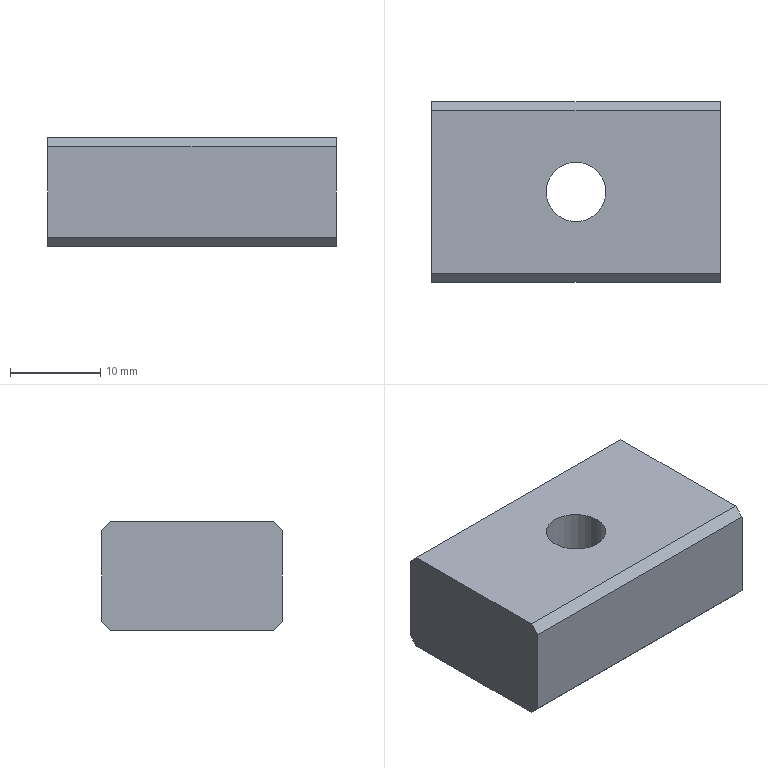Component | NX | LOCATING_KEY | 1 solid | 13 faces | box 32 x 20 x 12 mm | volume 6792 mm3 | plane 11 | cylinder 2 | commonest cylinder face diameters 6.6 x1 11 x1
STEP:
#1=CARTESIAN_POINT('',(0.,0.,0.));
#2=DIRECTION('',(0.,0.,1.));
#3=DIRECTION('',(1.,0.,0.));
#4=AXIS2_PLACEMENT_3D('',#1,#2,#3);
#5=CARTESIAN_POINT('',(250.,10.,-50.));
#6=VERTEX_POINT('',#5);
#7=CARTESIAN_POINT('',(250.,10.,-60.));
#8=VERTEX_POINT('',#7);
#9=CARTESIAN_POINT('',(250.,10.,-49.));
#10=DIRECTION('',(0.,0.,-1.));
#11=VECTOR('',#10,1.);
#12=LINE('',#9,#11);
#13=CARTESIAN_POINT('',(250.,10.,-49.));
#14=DIRECTION('',(1.,0.,0.));
#15=DIRECTION('',(0.,0.,-1.));
#16=AXIS2_PLACEMENT_3D('',#13,#14,#15);
#17=PLANE('',#16);
#18=CARTESIAN_POINT('',(0.,0.));
#19=DIRECTION('',(1.,0.));
#20=VECTOR('',#19,1.);
#21=LINE('',#18,#20);
#22=(GEOMETRIC_REPRESENTATION_CONTEXT(2)PARAMETRIC_REPRESENTATION_CONTEXT()REPRESENTATION_CONTEXT('',''));
#23=DEFINITIONAL_REPRESENTATION('',(#21),#22);
#24=PCURVE('',#17,#23);
#25=CARTESIAN_POINT('',(282.,10.,-49.));
#26=DIRECTION('',(0.,-1.,0.));
#27=DIRECTION('',(0.,0.,-1.));
#28=AXIS2_PLACEMENT_3D('',#25,#26,#27);
#29=PLANE('',#28);
#30=CARTESIAN_POINT('',(0.,-32.));
#31=DIRECTION('',(1.,0.));
#32=VECTOR('',#31,1.);
#33=LINE('',#30,#32);
#34=(GEOMETRIC_REPRESENTATION_CONTEXT(2)PARAMETRIC_REPRESENTATION_CONTEXT()REPRESENTATION_CONTEXT('',''));
#35=DEFINITIONAL_REPRESENTATION('',(#33),#34);
#36=PCURVE('',#29,#35);
#37=SURFACE_CURVE('',#12,(#24,#36),.PCURVE_S1.);
#38=EDGE_CURVE('',#6,#8,#37,.T.);
#39=ORIENTED_EDGE('',*,*,#38,.T.);
#40=CARTESIAN_POINT('',(250.,9.,-61.));
#41=VERTEX_POINT('',#40);
#42=CARTESIAN_POINT('',(250.,10.,-60.));
#43=DIRECTION('',(0.,-0.7071,-0.7071));
#44=VECTOR('',#43,1.);
#45=LINE('',#42,#44);
#46=CARTESIAN_POINT('',(11.,0.));
#47=DIRECTION('',(0.7071,-0.7071));
#48=VECTOR('',#47,1.);
#49=LINE('',#46,#48);
#50=(GEOMETRIC_REPRESENTATION_CONTEXT(2)PARAMETRIC_REPRESENTATION_CONTEXT()REPRESENTATION_CONTEXT('',''));
#51=DEFINITIONAL_REPRESENTATION('',(#49),#50);
#52=PCURVE('',#17,#51);
#53=CARTESIAN_POINT('',(282.,10.,-60.));
#54=DIRECTION('',(0.,-0.7071,0.7071));
#55=DIRECTION('',(-1.,0.,0.));
#56=AXIS2_PLACEMENT_3D('',#53,#54,#55);
#57=PLANE('',#56);
#58=CARTESIAN_POINT('',(32.,0.));
#59=DIRECTION('',(0.,1.));
#60=VECTOR('',#59,1.);
#61=LINE('',#58,#60);
#62=(GEOMETRIC_REPRESENTATION_CONTEXT(2)PARAMETRIC_REPRESENTATION_CONTEXT()REPRESENTATION_CONTEXT('',''));
#63=DEFINITIONAL_REPRESENTATION('',(#61),#62);
#64=PCURVE('',#57,#63);
#65=SURFACE_CURVE('',#45,(#52,#64),.PCURVE_S1.);
#66=EDGE_CURVE('',#8,#41,#65,.T.);
#67=ORIENTED_EDGE('',*,*,#66,.T.);
#68=CARTESIAN_POINT('',(250.,-9.,-61.));
#69=VERTEX_POINT('',#68);
#70=CARTESIAN_POINT('',(250.,10.,-61.));
#71=DIRECTION('',(0.,-1.,0.));
#72=VECTOR('',#71,1.);
#73=LINE('',#70,#72);
#74=CARTESIAN_POINT('',(12.,0.));
#75=DIRECTION('',(0.,-1.));
#76=VECTOR('',#75,1.);
#77=LINE('',#74,#76);
#78=(GEOMETRIC_REPRESENTATION_CONTEXT(2)PARAMETRIC_REPRESENTATION_CONTEXT()REPRESENTATION_CONTEXT('',''));
#79=DEFINITIONAL_REPRESENTATION('',(#77),#78);
#80=PCURVE('',#17,#79);
#81=CARTESIAN_POINT('',(266.,-0.,-61.));
#82=DIRECTION('',(0.,0.,1.));
#83=DIRECTION('',(1.,0.,0.));
#84=AXIS2_PLACEMENT_3D('',#81,#82,#83);
#85=PLANE('',#84);
#86=CARTESIAN_POINT('',(-16.,10.));
#87=DIRECTION('',(0.,-1.));
#88=VECTOR('',#87,1.);
#89=LINE('',#86,#88);
#90=(GEOMETRIC_REPRESENTATION_CONTEXT(2)PARAMETRIC_REPRESENTATION_CONTEXT()REPRESENTATION_CONTEXT('',''));
#91=DEFINITIONAL_REPRESENTATION('',(#89),#90);
#92=PCURVE('',#85,#91);
#93=SURFACE_CURVE('',#73,(#80,#92),.PCURVE_S1.);
#94=EDGE_CURVE('',#41,#69,#93,.T.);
#95=ORIENTED_EDGE('',*,*,#94,.T.);
#96=CARTESIAN_POINT('',(250.,-10.,-60.));
#97=VERTEX_POINT('',#96);
#98=CARTESIAN_POINT('',(250.,-10.,-60.));
#99=DIRECTION('',(0.,-0.7071,0.7071));
#100=VECTOR('',#99,1.);
#101=LINE('',#98,#100);
#102=CARTESIAN_POINT('',(11.,-20.));
#103=DIRECTION('',(-0.7071,-0.7071));
#104=VECTOR('',#103,1.);
#105=LINE('',#102,#104);
#106=(GEOMETRIC_REPRESENTATION_CONTEXT(2)PARAMETRIC_REPRESENTATION_CONTEXT()REPRESENTATION_CONTEXT('',''));
#107=DEFINITIONAL_REPRESENTATION('',(#105),#106);
#108=PCURVE('',#17,#107);
#109=CARTESIAN_POINT('',(250.,-10.,-60.));
#110=DIRECTION('',(0.,0.7071,0.7071));
#111=DIRECTION('',(1.,0.,0.));
#112=AXIS2_PLACEMENT_3D('',#109,#110,#111);
#113=PLANE('',#112);
#114=CARTESIAN_POINT('',(0.,0.));
#115=DIRECTION('',(0.,-1.));
#116=VECTOR('',#115,1.);
#117=LINE('',#114,#116);
#118=(GEOMETRIC_REPRESENTATION_CONTEXT(2)PARAMETRIC_REPRESENTATION_CONTEXT()REPRESENTATION_CONTEXT('',''));
#119=DEFINITIONAL_REPRESENTATION('',(#117),#118);
#120=PCURVE('',#113,#119);
#121=SURFACE_CURVE('',#101,(#108,#120),.PCURVE_S1.);
#122=EDGE_CURVE('',#69,#97,#121,.T.);
#123=ORIENTED_EDGE('',*,*,#122,.T.);
#124=CARTESIAN_POINT('',(250.,-10.,-50.));
#125=VERTEX_POINT('',#124);
#126=CARTESIAN_POINT('',(250.,-10.,-49.));
#127=DIRECTION('',(0.,0.,-1.));
#128=VECTOR('',#127,1.);
#129=LINE('',#126,#128);
#130=CARTESIAN_POINT('',(0.,-20.));
#131=DIRECTION('',(1.,0.));
#132=VECTOR('',#131,1.);
#133=LINE('',#130,#132);
#134=(GEOMETRIC_REPRESENTATION_CONTEXT(2)PARAMETRIC_REPRESENTATION_CONTEXT()REPRESENTATION_CONTEXT('',''));
#135=DEFINITIONAL_REPRESENTATION('',(#133),#134);
#136=PCURVE('',#17,#135);
#137=CARTESIAN_POINT('',(250.,-10.,-49.));
#138=DIRECTION('',(0.,1.,0.));
#139=DIRECTION('',(0.,0.,1.));
#140=AXIS2_PLACEMENT_3D('',#137,#138,#139);
#141=PLANE('',#140);
#142=CARTESIAN_POINT('',(0.,0.));
#143=DIRECTION('',(-1.,0.));
#144=VECTOR('',#143,1.);
#145=LINE('',#142,#144);
#146=(GEOMETRIC_REPRESENTATION_CONTEXT(2)PARAMETRIC_REPRESENTATION_CONTEXT()REPRESENTATION_CONTEXT('',''));
#147=DEFINITIONAL_REPRESENTATION('',(#145),#146);
#148=PCURVE('',#141,#147);
#149=SURFACE_CURVE('',#129,(#136,#148),.PCURVE_S1.);
#150=EDGE_CURVE('',#125,#97,#149,.T.);
#151=ORIENTED_EDGE('',*,*,#150,.F.);
#152=CARTESIAN_POINT('',(250.,-9.,-49.));
#153=VERTEX_POINT('',#152);
#154=CARTESIAN_POINT('',(250.,-9.,-49.));
#155=DIRECTION('',(0.,0.7071,0.7071));
#156=VECTOR('',#155,1.);
#157=LINE('',#154,#156);
#158=CARTESIAN_POINT('',(0.,-19.));
#159=DIRECTION('',(-0.7071,0.7071));
#160=VECTOR('',#159,1.);
#161=LINE('',#158,#160);
#162=(GEOMETRIC_REPRESENTATION_CONTEXT(2)PARAMETRIC_REPRESENTATION_CONTEXT()REPRESENTATION_CONTEXT('',''));
#163=DEFINITIONAL_REPRESENTATION('',(#161),#162);
#164=PCURVE('',#17,#163);
#165=CARTESIAN_POINT('',(266.,-9.,-49.));
#166=DIRECTION('',(0.,-0.7071,0.7071));
#167=DIRECTION('',(-1.,0.,0.));
#168=AXIS2_PLACEMENT_3D('',#165,#166,#167);
#169=PLANE('',#168);
#170=CARTESIAN_POINT('',(16.,0.));
#171=DIRECTION('',(0.,-1.));
#172=VECTOR('',#171,1.);
#173=LINE('',#170,#172);
#174=(GEOMETRIC_REPRESENTATION_CONTEXT(2)PARAMETRIC_REPRESENTATION_CONTEXT()REPRESENTATION_CONTEXT('',''));
#175=DEFINITIONAL_REPRESENTATION('',(#173),#174);
#176=PCURVE('',#169,#175);
#177=SURFACE_CURVE('',#157,(#164,#176),.PCURVE_S1.);
#178=EDGE_CURVE('',#125,#153,#177,.T.);
#179=ORIENTED_EDGE('',*,*,#178,.T.);
#180=CARTESIAN_POINT('',(250.,9.,-49.));
#181=VERTEX_POINT('',#180);
#182=CARTESIAN_POINT('',(250.,10.,-49.));
#183=DIRECTION('',(0.,-1.,0.));
#184=VECTOR('',#183,1.);
#185=LINE('',#182,#184);
#186=CARTESIAN_POINT('',(0.,0.));
#187=DIRECTION('',(0.,-1.));
#188=VECTOR('',#187,1.);
#189=LINE('',#186,#188);
#190=(GEOMETRIC_REPRESENTATION_CONTEXT(2)PARAMETRIC_REPRESENTATION_CONTEXT()REPRESENTATION_CONTEXT('',''));
#191=DEFINITIONAL_REPRESENTATION('',(#189),#190);
#192=PCURVE('',#17,#191);
#193=CARTESIAN_POINT('',(266.,-0.,-49.));
#194=DIRECTION('',(0.,0.,1.));
#195=DIRECTION('',(1.,0.,0.));
#196=AXIS2_PLACEMENT_3D('',#193,#194,#195);
#197=PLANE('',#196);
#198=CARTESIAN_POINT('',(-16.,10.));
#199=DIRECTION('',(0.,-1.));
#200=VECTOR('',#199,1.);
#201=LINE('',#198,#200);
#202=(GEOMETRIC_REPRESENTATION_CONTEXT(2)PARAMETRIC_REPRESENTATION_CONTEXT()REPRESENTATION_CONTEXT('',''));
#203=DEFINITIONAL_REPRESENTATION('',(#201),#202);
#204=PCURVE('',#197,#203);
#205=SURFACE_CURVE('',#185,(#192,#204),.PCURVE_S1.);
#206=EDGE_CURVE('',#181,#153,#205,.T.);
#207=ORIENTED_EDGE('',*,*,#206,.F.);
#208=CARTESIAN_POINT('',(250.,9.,-49.));
#209=DIRECTION('',(0.,0.7071,-0.7071));
#210=VECTOR('',#209,1.);
#211=LINE('',#208,#210);
#212=CARTESIAN_POINT('',(0.,-1.));
#213=DIRECTION('',(0.7071,0.7071));
#214=VECTOR('',#213,1.);
#215=LINE('',#212,#214);
#216=(GEOMETRIC_REPRESENTATION_CONTEXT(2)PARAMETRIC_REPRESENTATION_CONTEXT()REPRESENTATION_CONTEXT('',''));
#217=DEFINITIONAL_REPRESENTATION('',(#215),#216);
#218=PCURVE('',#17,#217);
#219=CARTESIAN_POINT('',(266.,9.,-49.));
#220=DIRECTION('',(0.,0.7071,0.7071));
#221=DIRECTION('',(1.,0.,0.));
#222=AXIS2_PLACEMENT_3D('',#219,#220,#221);
#223=PLANE('',#222);
#224=CARTESIAN_POINT('',(-16.,0.));
#225=DIRECTION('',(0.,1.));
#226=VECTOR('',#225,1.);
#227=LINE('',#224,#226);
#228=(GEOMETRIC_REPRESENTATION_CONTEXT(2)PARAMETRIC_REPRESENTATION_CONTEXT()REPRESENTATION_CONTEXT('',''));
#229=DEFINITIONAL_REPRESENTATION('',(#227),#228);
#230=PCURVE('',#223,#229);
#231=SURFACE_CURVE('',#211,(#218,#230),.PCURVE_S1.);
#232=EDGE_CURVE('',#181,#6,#231,.T.);
#233=ORIENTED_EDGE('',*,*,#232,.T.);
#234=EDGE_LOOP('',(#39,#67,#95,#123,#151,#179,#207,#233));
#235=FACE_BOUND('',#234,.T.);
#236=ADVANCED_FACE('',(#235),#17,.F.);
#237=ORIENTED_EDGE('',*,*,#150,.T.);
#238=CARTESIAN_POINT('',(282.,-10.,-60.));
#239=VERTEX_POINT('',#238);
#240=CARTESIAN_POINT('',(250.,-10.,-60.));
#241=DIRECTION('',(1.,0.,0.));
#242=VECTOR('',#241,1.);
#243=LINE('',#240,#242);
#244=CARTESIAN_POINT('',(-11.,0.));
#245=DIRECTION('',(0.,1.));
#246=VECTOR('',#245,1.);
#247=LINE('',#244,#246);
#248=(GEOMETRIC_REPRESENTATION_CONTEXT(2)PARAMETRIC_REPRESENTATION_CONTEXT()REPRESENTATION_CONTEXT('',''));
#249=DEFINITIONAL_REPRESENTATION('',(#247),#248);
#250=PCURVE('',#141,#249);
#251=CARTESIAN_POINT('',(0.,0.));
#252=DIRECTION('',(1.,0.));
#253=VECTOR('',#252,1.);
#254=LINE('',#251,#253);
#255=(GEOMETRIC_REPRESENTATION_CONTEXT(2)PARAMETRIC_REPRESENTATION_CONTEXT()REPRESENTATION_CONTEXT('',''));
#256=DEFINITIONAL_REPRESENTATION('',(#254),#255);
#257=PCURVE('',#113,#256);
#258=SURFACE_CURVE('',#243,(#250,#257),.PCURVE_S1.);
#259=EDGE_CURVE('',#97,#239,#258,.T.);
#260=ORIENTED_EDGE('',*,*,#259,.T.);
#261=CARTESIAN_POINT('',(282.,-10.,-50.));
#262=VERTEX_POINT('',#261);
#263=CARTESIAN_POINT('',(282.,-10.,-49.));
#264=DIRECTION('',(0.,0.,-1.));
#265=VECTOR('',#264,1.);
#266=LINE('',#263,#265);
#267=CARTESIAN_POINT('',(0.,32.));
#268=DIRECTION('',(-1.,0.));
#269=VECTOR('',#268,1.);
#270=LINE('',#267,#269);
#271=(GEOMETRIC_REPRESENTATION_CONTEXT(2)PARAMETRIC_REPRESENTATION_CONTEXT()REPRESENTATION_CONTEXT('',''));
#272=DEFINITIONAL_REPRESENTATION('',(#270),#271);
#273=PCURVE('',#141,#272);
#274=CARTESIAN_POINT('',(282.,-10.,-49.));
#275=DIRECTION('',(-1.,0.,0.));
#276=DIRECTION('',(0.,0.,1.));
#277=AXIS2_PLACEMENT_3D('',#274,#275,#276);
#278=PLANE('',#277);
#279=CARTESIAN_POINT('',(0.,0.));
#280=DIRECTION('',(-1.,0.));
#281=VECTOR('',#280,1.);
#282=LINE('',#279,#281);
#283=(GEOMETRIC_REPRESENTATION_CONTEXT(2)PARAMETRIC_REPRESENTATION_CONTEXT()REPRESENTATION_CONTEXT('',''));
#284=DEFINITIONAL_REPRESENTATION('',(#282),#283);
#285=PCURVE('',#278,#284);
#286=SURFACE_CURVE('',#266,(#273,#285),.PCURVE_S1.);
#287=EDGE_CURVE('',#262,#239,#286,.T.);
#288=ORIENTED_EDGE('',*,*,#287,.F.);
#289=CARTESIAN_POINT('',(250.,-10.,-50.));
#290=DIRECTION('',(-1.,0.,0.));
#291=VECTOR('',#290,1.);
#292=LINE('',#289,#291);
#293=CARTESIAN_POINT('',(-1.,0.));
#294=DIRECTION('',(0.,-1.));
#295=VECTOR('',#294,1.);
#296=LINE('',#293,#295);
#297=(GEOMETRIC_REPRESENTATION_CONTEXT(2)PARAMETRIC_REPRESENTATION_CONTEXT()REPRESENTATION_CONTEXT('',''));
#298=DEFINITIONAL_REPRESENTATION('',(#296),#297);
#299=PCURVE('',#141,#298);
#300=CARTESIAN_POINT('',(16.,1.414));
#301=DIRECTION('',(1.,0.));
#302=VECTOR('',#301,1.);
#303=LINE('',#300,#302);
#304=(GEOMETRIC_REPRESENTATION_CONTEXT(2)PARAMETRIC_REPRESENTATION_CONTEXT()REPRESENTATION_CONTEXT('',''));
#305=DEFINITIONAL_REPRESENTATION('',(#303),#304);
#306=PCURVE('',#169,#305);
#307=SURFACE_CURVE('',#292,(#299,#306),.PCURVE_S1.);
#308=EDGE_CURVE('',#262,#125,#307,.T.);
#309=ORIENTED_EDGE('',*,*,#308,.T.);
#310=EDGE_LOOP('',(#237,#260,#288,#309));
#311=FACE_BOUND('',#310,.T.);
#312=ADVANCED_FACE('',(#311),#141,.F.);
#313=CARTESIAN_POINT('',(282.,-9.,-61.));
#314=VERTEX_POINT('',#313);
#315=CARTESIAN_POINT('',(282.,9.,-61.));
#316=VERTEX_POINT('',#315);
#317=CARTESIAN_POINT('',(282.,-10.,-61.));
#318=DIRECTION('',(0.,1.,0.));
#319=VECTOR('',#318,1.);
#320=LINE('',#317,#319);
#321=CARTESIAN_POINT('',(-12.,0.));
#322=DIRECTION('',(0.,1.));
#323=VECTOR('',#322,1.);
#324=LINE('',#321,#323);
#325=(GEOMETRIC_REPRESENTATION_CONTEXT(2)PARAMETRIC_REPRESENTATION_CONTEXT()REPRESENTATION_CONTEXT('',''));
#326=DEFINITIONAL_REPRESENTATION('',(#324),#325);
#327=PCURVE('',#278,#326);
#328=CARTESIAN_POINT('',(16.,-10.));
#329=DIRECTION('',(0.,1.));
#330=VECTOR('',#329,1.);
#331=LINE('',#328,#330);
#332=(GEOMETRIC_REPRESENTATION_CONTEXT(2)PARAMETRIC_REPRESENTATION_CONTEXT()REPRESENTATION_CONTEXT('',''));
#333=DEFINITIONAL_REPRESENTATION('',(#331),#332);
#334=PCURVE('',#85,#333);
#335=SURFACE_CURVE('',#320,(#327,#334),.PCURVE_S1.);
#336=EDGE_CURVE('',#314,#316,#335,.T.);
#337=ORIENTED_EDGE('',*,*,#336,.T.);
#338=CARTESIAN_POINT('',(282.,10.,-60.));
#339=VERTEX_POINT('',#338);
#340=CARTESIAN_POINT('',(282.,10.,-60.));
#341=DIRECTION('',(0.,0.7071,0.7071));
#342=VECTOR('',#341,1.);
#343=LINE('',#340,#342);
#344=CARTESIAN_POINT('',(-11.,20.));
#345=DIRECTION('',(0.7071,0.7071));
#346=VECTOR('',#345,1.);
#347=LINE('',#344,#346);
#348=(GEOMETRIC_REPRESENTATION_CONTEXT(2)PARAMETRIC_REPRESENTATION_CONTEXT()REPRESENTATION_CONTEXT('',''));
#349=DEFINITIONAL_REPRESENTATION('',(#347),#348);
#350=PCURVE('',#278,#349);
#351=CARTESIAN_POINT('',(0.,0.));
#352=DIRECTION('',(0.,-1.));
#353=VECTOR('',#352,1.);
#354=LINE('',#351,#353);
#355=(GEOMETRIC_REPRESENTATION_CONTEXT(2)PARAMETRIC_REPRESENTATION_CONTEXT()REPRESENTATION_CONTEXT('',''));
#356=DEFINITIONAL_REPRESENTATION('',(#354),#355);
#357=PCURVE('',#57,#356);
#358=SURFACE_CURVE('',#343,(#350,#357),.PCURVE_S1.);
#359=EDGE_CURVE('',#316,#339,#358,.T.);
#360=ORIENTED_EDGE('',*,*,#359,.T.);
#361=CARTESIAN_POINT('',(282.,10.,-50.));
#362=VERTEX_POINT('',#361);
#363=CARTESIAN_POINT('',(282.,10.,-49.));
#364=DIRECTION('',(0.,0.,-1.));
#365=VECTOR('',#364,1.);
#366=LINE('',#363,#365);
#367=CARTESIAN_POINT('',(0.,20.));
#368=DIRECTION('',(-1.,0.));
#369=VECTOR('',#368,1.);
#370=LINE('',#367,#369);
#371=(GEOMETRIC_REPRESENTATION_CONTEXT(2)PARAMETRIC_REPRESENTATION_CONTEXT()REPRESENTATION_CONTEXT('',''));
#372=DEFINITIONAL_REPRESENTATION('',(#370),#371);
#373=PCURVE('',#278,#372);
#374=CARTESIAN_POINT('',(0.,0.));
#375=DIRECTION('',(1.,0.));
#376=VECTOR('',#375,1.);
#377=LINE('',#374,#376);
#378=(GEOMETRIC_REPRESENTATION_CONTEXT(2)PARAMETRIC_REPRESENTATION_CONTEXT()REPRESENTATION_CONTEXT('',''));
#379=DEFINITIONAL_REPRESENTATION('',(#377),#378);
#380=PCURVE('',#29,#379);
#381=SURFACE_CURVE('',#366,(#373,#380),.PCURVE_S1.);
#382=EDGE_CURVE('',#362,#339,#381,.T.);
#383=ORIENTED_EDGE('',*,*,#382,.F.);
#384=CARTESIAN_POINT('',(282.,9.,-49.));
#385=VERTEX_POINT('',#384);
#386=CARTESIAN_POINT('',(282.,9.,-49.));
#387=DIRECTION('',(0.,-0.7071,0.7071));
#388=VECTOR('',#387,1.);
#389=LINE('',#386,#388);
#390=CARTESIAN_POINT('',(0.,19.));
#391=DIRECTION('',(0.7071,-0.7071));
#392=VECTOR('',#391,1.);
#393=LINE('',#390,#392);
#394=(GEOMETRIC_REPRESENTATION_CONTEXT(2)PARAMETRIC_REPRESENTATION_CONTEXT()REPRESENTATION_CONTEXT('',''));
#395=DEFINITIONAL_REPRESENTATION('',(#393),#394);
#396=PCURVE('',#278,#395);
#397=CARTESIAN_POINT('',(16.,0.));
#398=DIRECTION('',(0.,-1.));
#399=VECTOR('',#398,1.);
#400=LINE('',#397,#399);
#401=(GEOMETRIC_REPRESENTATION_CONTEXT(2)PARAMETRIC_REPRESENTATION_CONTEXT()REPRESENTATION_CONTEXT('',''));
#402=DEFINITIONAL_REPRESENTATION('',(#400),#401);
#403=PCURVE('',#223,#402);
#404=SURFACE_CURVE('',#389,(#396,#403),.PCURVE_S1.);
#405=EDGE_CURVE('',#362,#385,#404,.T.);
#406=ORIENTED_EDGE('',*,*,#405,.T.);
#407=CARTESIAN_POINT('',(282.,-9.,-49.));
#408=VERTEX_POINT('',#407);
#409=CARTESIAN_POINT('',(282.,-10.,-49.));
#410=DIRECTION('',(0.,1.,0.));
#411=VECTOR('',#410,1.);
#412=LINE('',#409,#411);
#413=CARTESIAN_POINT('',(0.,0.));
#414=DIRECTION('',(0.,1.));
#415=VECTOR('',#414,1.);
#416=LINE('',#413,#415);
#417=(GEOMETRIC_REPRESENTATION_CONTEXT(2)PARAMETRIC_REPRESENTATION_CONTEXT()REPRESENTATION_CONTEXT('',''));
#418=DEFINITIONAL_REPRESENTATION('',(#416),#417);
#419=PCURVE('',#278,#418);
#420=CARTESIAN_POINT('',(16.,-10.));
#421=DIRECTION('',(0.,1.));
#422=VECTOR('',#421,1.);
#423=LINE('',#420,#422);
#424=(GEOMETRIC_REPRESENTATION_CONTEXT(2)PARAMETRIC_REPRESENTATION_CONTEXT()REPRESENTATION_CONTEXT('',''));
#425=DEFINITIONAL_REPRESENTATION('',(#423),#424);
#426=PCURVE('',#197,#425);
#427=SURFACE_CURVE('',#412,(#419,#426),.PCURVE_S1.);
#428=EDGE_CURVE('',#408,#385,#427,.T.);
#429=ORIENTED_EDGE('',*,*,#428,.F.);
#430=CARTESIAN_POINT('',(282.,-9.,-49.));
#431=DIRECTION('',(0.,-0.7071,-0.7071));
#432=VECTOR('',#431,1.);
#433=LINE('',#430,#432);
#434=CARTESIAN_POINT('',(0.,1.));
#435=DIRECTION('',(-0.7071,-0.7071));
#436=VECTOR('',#435,1.);
#437=LINE('',#434,#436);
#438=(GEOMETRIC_REPRESENTATION_CONTEXT(2)PARAMETRIC_REPRESENTATION_CONTEXT()REPRESENTATION_CONTEXT('',''));
#439=DEFINITIONAL_REPRESENTATION('',(#437),#438);
#440=PCURVE('',#278,#439);
#441=CARTESIAN_POINT('',(-16.,0.));
#442=DIRECTION('',(0.,1.));
#443=VECTOR('',#442,1.);
#444=LINE('',#441,#443);
#445=(GEOMETRIC_REPRESENTATION_CONTEXT(2)PARAMETRIC_REPRESENTATION_CONTEXT()REPRESENTATION_CONTEXT('',''));
#446=DEFINITIONAL_REPRESENTATION('',(#444),#445);
#447=PCURVE('',#169,#446);
#448=SURFACE_CURVE('',#433,(#440,#447),.PCURVE_S1.);
#449=EDGE_CURVE('',#408,#262,#448,.T.);
#450=ORIENTED_EDGE('',*,*,#449,.T.);
#451=ORIENTED_EDGE('',*,*,#287,.T.);
#452=CARTESIAN_POINT('',(282.,-10.,-60.));
#453=DIRECTION('',(0.,0.7071,-0.7071));
#454=VECTOR('',#453,1.);
#455=LINE('',#452,#454);
#456=CARTESIAN_POINT('',(-11.,0.));
#457=DIRECTION('',(-0.7071,0.7071));
#458=VECTOR('',#457,1.);
#459=LINE('',#456,#458);
#460=(GEOMETRIC_REPRESENTATION_CONTEXT(2)PARAMETRIC_REPRESENTATION_CONTEXT()REPRESENTATION_CONTEXT('',''));
#461=DEFINITIONAL_REPRESENTATION('',(#459),#460);
#462=PCURVE('',#278,#461);
#463=CARTESIAN_POINT('',(32.,0.));
#464=DIRECTION('',(0.,1.));
#465=VECTOR('',#464,1.);
#466=LINE('',#463,#465);
#467=(GEOMETRIC_REPRESENTATION_CONTEXT(2)PARAMETRIC_REPRESENTATION_CONTEXT()REPRESENTATION_CONTEXT('',''));
#468=DEFINITIONAL_REPRESENTATION('',(#466),#467);
#469=PCURVE('',#113,#468);
#470=SURFACE_CURVE('',#455,(#462,#469),.PCURVE_S1.);
#471=EDGE_CURVE('',#239,#314,#470,.T.);
#472=ORIENTED_EDGE('',*,*,#471,.T.);
#473=EDGE_LOOP('',(#337,#360,#383,#406,#429,#450,#451,#472));
#474=FACE_BOUND('',#473,.T.);
#475=ADVANCED_FACE('',(#474),#278,.F.);
#476=ORIENTED_EDGE('',*,*,#382,.T.);
#477=CARTESIAN_POINT('',(282.,10.,-60.));
#478=DIRECTION('',(-1.,0.,0.));
#479=VECTOR('',#478,1.);
#480=LINE('',#477,#479);
#481=CARTESIAN_POINT('',(11.,0.));
#482=DIRECTION('',(0.,-1.));
#483=VECTOR('',#482,1.);
#484=LINE('',#481,#483);
#485=(GEOMETRIC_REPRESENTATION_CONTEXT(2)PARAMETRIC_REPRESENTATION_CONTEXT()REPRESENTATION_CONTEXT('',''));
#486=DEFINITIONAL_REPRESENTATION('',(#484),#485);
#487=PCURVE('',#29,#486);
#488=CARTESIAN_POINT('',(0.,0.));
#489=DIRECTION('',(1.,0.));
#490=VECTOR('',#489,1.);
#491=LINE('',#488,#490);
#492=(GEOMETRIC_REPRESENTATION_CONTEXT(2)PARAMETRIC_REPRESENTATION_CONTEXT()REPRESENTATION_CONTEXT('',''));
#493=DEFINITIONAL_REPRESENTATION('',(#491),#492);
#494=PCURVE('',#57,#493);
#495=SURFACE_CURVE('',#480,(#487,#494),.PCURVE_S1.);
#496=EDGE_CURVE('',#339,#8,#495,.T.);
#497=ORIENTED_EDGE('',*,*,#496,.T.);
#498=ORIENTED_EDGE('',*,*,#38,.F.);
#499=CARTESIAN_POINT('',(282.,10.,-50.));
#500=DIRECTION('',(1.,0.,0.));
#501=VECTOR('',#500,1.);
#502=LINE('',#499,#501);
#503=CARTESIAN_POINT('',(1.,0.));
#504=DIRECTION('',(0.,1.));
#505=VECTOR('',#504,1.);
#506=LINE('',#503,#505);
#507=(GEOMETRIC_REPRESENTATION_CONTEXT(2)PARAMETRIC_REPRESENTATION_CONTEXT()REPRESENTATION_CONTEXT('',''));
#508=DEFINITIONAL_REPRESENTATION('',(#506),#507);
#509=PCURVE('',#29,#508);
#510=CARTESIAN_POINT('',(16.,1.414));
#511=DIRECTION('',(1.,0.));
#512=VECTOR('',#511,1.);
#513=LINE('',#510,#512);
#514=(GEOMETRIC_REPRESENTATION_CONTEXT(2)PARAMETRIC_REPRESENTATION_CONTEXT()REPRESENTATION_CONTEXT('',''));
#515=DEFINITIONAL_REPRESENTATION('',(#513),#514);
#516=PCURVE('',#223,#515);
#517=SURFACE_CURVE('',#502,(#509,#516),.PCURVE_S1.);
#518=EDGE_CURVE('',#6,#362,#517,.T.);
#519=ORIENTED_EDGE('',*,*,#518,.T.);
#520=EDGE_LOOP('',(#476,#497,#498,#519));
#521=FACE_BOUND('',#520,.T.);
#522=ADVANCED_FACE('',(#521),#29,.F.);
#523=CARTESIAN_POINT('',(269.3,-0.,-49.));
#524=VERTEX_POINT('',#523);
#525=CARTESIAN_POINT('',(266.,-0.,-49.));
#526=DIRECTION('',(0.,0.,1.));
#527=DIRECTION('',(1.,0.,0.));
#528=AXIS2_PLACEMENT_3D('',#525,#526,#527);
#529=CIRCLE('',#528,3.3);
#530=CARTESIAN_POINT('',(0.,0.));
#531=DIRECTION('',(1.,0.));
#532=AXIS2_PLACEMENT_2D('',#530,#531);
#533=CIRCLE('',#532,3.3);
#534=(GEOMETRIC_REPRESENTATION_CONTEXT(2)PARAMETRIC_REPRESENTATION_CONTEXT()REPRESENTATION_CONTEXT('',''));
#535=DEFINITIONAL_REPRESENTATION('',(#533),#534);
#536=PCURVE('',#197,#535);
#537=CARTESIAN_POINT('',(266.,-0.,-33.221));
#538=DIRECTION('',(0.,0.,1.));
#539=DIRECTION('',(1.,0.,0.));
#540=AXIS2_PLACEMENT_3D('',#537,#538,#539);
#541=CYLINDRICAL_SURFACE('',#540,3.3);
#542=CARTESIAN_POINT('',(0.,-15.779));
#543=DIRECTION('',(1.,0.));
#544=VECTOR('',#543,1.);
#545=LINE('',#542,#544);
#546=(GEOMETRIC_REPRESENTATION_CONTEXT(2)PARAMETRIC_REPRESENTATION_CONTEXT()REPRESENTATION_CONTEXT('',''));
#547=DEFINITIONAL_REPRESENTATION('',(#545),#546);
#548=PCURVE('',#541,#547);
#549=SURFACE_CURVE('',#529,(#536,#548),.PCURVE_S1.);
#550=EDGE_CURVE('',#524,#524,#549,.T.);
#551=ORIENTED_EDGE('',*,*,#550,.F.);
#552=EDGE_LOOP('',(#551));
#553=FACE_BOUND('',#552,.T.);
#554=ORIENTED_EDGE('',*,*,#206,.T.);
#555=CARTESIAN_POINT('',(282.,-9.,-49.));
#556=DIRECTION('',(1.,0.,0.));
#557=VECTOR('',#556,1.);
#558=LINE('',#555,#557);
#559=CARTESIAN_POINT('',(16.,-9.));
#560=DIRECTION('',(1.,0.));
#561=VECTOR('',#560,1.);
#562=LINE('',#559,#561);
#563=(GEOMETRIC_REPRESENTATION_CONTEXT(2)PARAMETRIC_REPRESENTATION_CONTEXT()REPRESENTATION_CONTEXT('',''));
#564=DEFINITIONAL_REPRESENTATION('',(#562),#563);
#565=PCURVE('',#197,#564);
#566=CARTESIAN_POINT('',(-16.,0.));
#567=DIRECTION('',(-1.,0.));
#568=VECTOR('',#567,1.);
#569=LINE('',#566,#568);
#570=(GEOMETRIC_REPRESENTATION_CONTEXT(2)PARAMETRIC_REPRESENTATION_CONTEXT()REPRESENTATION_CONTEXT('',''));
#571=DEFINITIONAL_REPRESENTATION('',(#569),#570);
#572=PCURVE('',#169,#571);
#573=SURFACE_CURVE('',#558,(#565,#572),.PCURVE_S1.);
#574=EDGE_CURVE('',#153,#408,#573,.T.);
#575=ORIENTED_EDGE('',*,*,#574,.T.);
#576=ORIENTED_EDGE('',*,*,#428,.T.);
#577=CARTESIAN_POINT('',(250.,9.,-49.));
#578=DIRECTION('',(-1.,0.,0.));
#579=VECTOR('',#578,1.);
#580=LINE('',#577,#579);
#581=CARTESIAN_POINT('',(-16.,9.));
#582=DIRECTION('',(-1.,0.));
#583=VECTOR('',#582,1.);
#584=LINE('',#581,#583);
#585=(GEOMETRIC_REPRESENTATION_CONTEXT(2)PARAMETRIC_REPRESENTATION_CONTEXT()REPRESENTATION_CONTEXT('',''));
#586=DEFINITIONAL_REPRESENTATION('',(#584),#585);
#587=PCURVE('',#197,#586);
#588=CARTESIAN_POINT('',(-16.,0.));
#589=DIRECTION('',(-1.,0.));
#590=VECTOR('',#589,1.);
#591=LINE('',#588,#590);
#592=(GEOMETRIC_REPRESENTATION_CONTEXT(2)PARAMETRIC_REPRESENTATION_CONTEXT()REPRESENTATION_CONTEXT('',''));
#593=DEFINITIONAL_REPRESENTATION('',(#591),#592);
#594=PCURVE('',#223,#593);
#595=SURFACE_CURVE('',#580,(#587,#594),.PCURVE_S1.);
#596=EDGE_CURVE('',#385,#181,#595,.T.);
#597=ORIENTED_EDGE('',*,*,#596,.T.);
#598=EDGE_LOOP('',(#554,#575,#576,#597));
#599=FACE_BOUND('',#598,.T.);
#600=ADVANCED_FACE('',(#553,#599),#197,.T.);
#601=CARTESIAN_POINT('',(271.5,-0.,-61.));
#602=VERTEX_POINT('',#601);
#603=CARTESIAN_POINT('',(266.,-0.,-61.));
#604=DIRECTION('',(0.,0.,1.));
#605=DIRECTION('',(1.,0.,0.));
#606=AXIS2_PLACEMENT_3D('',#603,#604,#605);
#607=CIRCLE('',#606,5.5);
#608=CARTESIAN_POINT('',(0.,0.));
#609=DIRECTION('',(1.,0.));
#610=AXIS2_PLACEMENT_2D('',#608,#609);
#611=CIRCLE('',#610,5.5);
#612=(GEOMETRIC_REPRESENTATION_CONTEXT(2)PARAMETRIC_REPRESENTATION_CONTEXT()REPRESENTATION_CONTEXT('',''));
#613=DEFINITIONAL_REPRESENTATION('',(#611),#612);
#614=PCURVE('',#85,#613);
#615=CARTESIAN_POINT('',(266.,-0.,-61.));
#616=DIRECTION('',(0.,0.,1.));
#617=DIRECTION('',(1.,0.,0.));
#618=AXIS2_PLACEMENT_3D('',#615,#616,#617);
#619=CYLINDRICAL_SURFACE('',#618,5.5);
#620=CARTESIAN_POINT('',(0.,0.));
#621=DIRECTION('',(1.,0.));
#622=VECTOR('',#621,1.);
#623=LINE('',#620,#622);
#624=(GEOMETRIC_REPRESENTATION_CONTEXT(2)PARAMETRIC_REPRESENTATION_CONTEXT()REPRESENTATION_CONTEXT('',''));
#625=DEFINITIONAL_REPRESENTATION('',(#623),#624);
#626=PCURVE('',#619,#625);
#627=SURFACE_CURVE('',#607,(#614,#626),.PCURVE_S1.);
#628=EDGE_CURVE('',#602,#602,#627,.T.);
#629=ORIENTED_EDGE('',*,*,#628,.T.);
#630=EDGE_LOOP('',(#629));
#631=FACE_BOUND('',#630,.T.);
#632=ORIENTED_EDGE('',*,*,#94,.F.);
#633=CARTESIAN_POINT('',(266.,9.,-61.));
#634=DIRECTION('',(1.,0.,0.));
#635=VECTOR('',#634,1.);
#636=LINE('',#633,#635);
#637=CARTESIAN_POINT('',(0.,9.));
#638=DIRECTION('',(1.,0.));
#639=VECTOR('',#638,1.);
#640=LINE('',#637,#639);
#641=(GEOMETRIC_REPRESENTATION_CONTEXT(2)PARAMETRIC_REPRESENTATION_CONTEXT()REPRESENTATION_CONTEXT('',''));
#642=DEFINITIONAL_REPRESENTATION('',(#640),#641);
#643=PCURVE('',#85,#642);
#644=CARTESIAN_POINT('',(16.,1.414));
#645=DIRECTION('',(-1.,0.));
#646=VECTOR('',#645,1.);
#647=LINE('',#644,#646);
#648=(GEOMETRIC_REPRESENTATION_CONTEXT(2)PARAMETRIC_REPRESENTATION_CONTEXT()REPRESENTATION_CONTEXT('',''));
#649=DEFINITIONAL_REPRESENTATION('',(#647),#648);
#650=PCURVE('',#57,#649);
#651=SURFACE_CURVE('',#636,(#643,#650),.PCURVE_S1.);
#652=EDGE_CURVE('',#41,#316,#651,.T.);
#653=ORIENTED_EDGE('',*,*,#652,.T.);
#654=ORIENTED_EDGE('',*,*,#336,.F.);
#655=CARTESIAN_POINT('',(266.,-9.,-61.));
#656=DIRECTION('',(-1.,0.,0.));
#657=VECTOR('',#656,1.);
#658=LINE('',#655,#657);
#659=CARTESIAN_POINT('',(0.,-9.));
#660=DIRECTION('',(-1.,0.));
#661=VECTOR('',#660,1.);
#662=LINE('',#659,#661);
#663=(GEOMETRIC_REPRESENTATION_CONTEXT(2)PARAMETRIC_REPRESENTATION_CONTEXT()REPRESENTATION_CONTEXT('',''));
#664=DEFINITIONAL_REPRESENTATION('',(#662),#663);
#665=PCURVE('',#85,#664);
#666=CARTESIAN_POINT('',(16.,1.414));
#667=DIRECTION('',(-1.,0.));
#668=VECTOR('',#667,1.);
#669=LINE('',#666,#668);
#670=(GEOMETRIC_REPRESENTATION_CONTEXT(2)PARAMETRIC_REPRESENTATION_CONTEXT()REPRESENTATION_CONTEXT('',''));
#671=DEFINITIONAL_REPRESENTATION('',(#669),#670);
#672=PCURVE('',#113,#671);
#673=SURFACE_CURVE('',#658,(#665,#672),.PCURVE_S1.);
#674=EDGE_CURVE('',#314,#69,#673,.T.);
#675=ORIENTED_EDGE('',*,*,#674,.T.);
#676=EDGE_LOOP('',(#632,#653,#654,#675));
#677=FACE_BOUND('',#676,.T.);
#678=ADVANCED_FACE('',(#631,#677),#85,.F.);
#679=ORIENTED_EDGE('',*,*,#550,.F.);
#680=CARTESIAN_POINT('',(269.3,-0.,-54.2));
#681=VERTEX_POINT('',#680);
#682=CARTESIAN_POINT('',(269.3,-0.,-54.2));
#683=CARTESIAN_POINT('',(269.3,-0.,-49.));
#684=B_SPLINE_CURVE_WITH_KNOTS('',1,(#682,#683),.UNSPECIFIED.,.F.,.F.,(2,2),(-20.979,-15.779),.PIECEWISE_BEZIER_KNOTS.);
#685=CARTESIAN_POINT('',(0.,0.));
#686=DIRECTION('',(0.,1.));
#687=VECTOR('',#686,1.);
#688=LINE('',#685,#687);
#689=(GEOMETRIC_REPRESENTATION_CONTEXT(2)PARAMETRIC_REPRESENTATION_CONTEXT()REPRESENTATION_CONTEXT('',''));
#690=DEFINITIONAL_REPRESENTATION('',(#688),#689);
#691=PCURVE('',#541,#690);
#692=CARTESIAN_POINT('',(6.283,0.));
#693=DIRECTION('',(0.,1.));
#694=VECTOR('',#693,1.);
#695=LINE('',#692,#694);
#696=(GEOMETRIC_REPRESENTATION_CONTEXT(2)PARAMETRIC_REPRESENTATION_CONTEXT()REPRESENTATION_CONTEXT('',''));
#697=DEFINITIONAL_REPRESENTATION('',(#695),#696);
#698=PCURVE('',#541,#697);
#699=SEAM_CURVE('',#684,(#691,#698),.PCURVE_S1.);
#700=EDGE_CURVE('',#681,#524,#699,.T.);
#701=ORIENTED_EDGE('',*,*,#700,.F.);
#702=CARTESIAN_POINT('',(266.,-0.,-54.2));
#703=DIRECTION('',(0.,0.,-1.));
#704=DIRECTION('',(1.,0.,0.));
#705=AXIS2_PLACEMENT_3D('',#702,#703,#704);
#706=CIRCLE('',#705,3.3);
#707=CARTESIAN_POINT('',(6.283,-20.979));
#708=DIRECTION('',(-1.,0.));
#709=VECTOR('',#708,1.);
#710=LINE('',#707,#709);
#711=(GEOMETRIC_REPRESENTATION_CONTEXT(2)PARAMETRIC_REPRESENTATION_CONTEXT()REPRESENTATION_CONTEXT('',''));
#712=DEFINITIONAL_REPRESENTATION('',(#710),#711);
#713=PCURVE('',#541,#712);
#714=CARTESIAN_POINT('',(266.,-0.,-54.2));
#715=DIRECTION('',(0.,0.,1.));
#716=DIRECTION('',(1.,0.,0.));
#717=AXIS2_PLACEMENT_3D('',#714,#715,#716);
#718=PLANE('',#717);
#719=CARTESIAN_POINT('',(3.3,0.));
#720=CARTESIAN_POINT('',(3.3,-5.716));
#721=CARTESIAN_POINT('',(-1.65,-2.858));
#722=CARTESIAN_POINT('',(-6.6,-0.));
#723=CARTESIAN_POINT('',(-1.65,2.858));
#724=CARTESIAN_POINT('',(3.3,5.716));
#725=CARTESIAN_POINT('',(3.3,0.));
#726=(BOUNDED_CURVE()B_SPLINE_CURVE(2,(#719,#720,#721,#722,#723,#724,#725),.UNSPECIFIED.,.T.,.F.)B_SPLINE_CURVE_WITH_KNOTS((1,2,2,2,2,1),(-2.094,0.,2.094,4.189,6.283,8.378),.UNSPECIFIED.)CURVE()GEOMETRIC_REPRESENTATION_ITEM()RATIONAL_B_SPLINE_CURVE((1.,0.5,1.,0.5,1.,0.5,1.))REPRESENTATION_ITEM(''));
#727=(GEOMETRIC_REPRESENTATION_CONTEXT(2)PARAMETRIC_REPRESENTATION_CONTEXT()REPRESENTATION_CONTEXT('',''));
#728=DEFINITIONAL_REPRESENTATION('',(#726),#727);
#729=PCURVE('',#718,#728);
#730=SURFACE_CURVE('',#706,(#713,#729),.PCURVE_S1.);
#731=EDGE_CURVE('',#681,#681,#730,.T.);
#732=ORIENTED_EDGE('',*,*,#731,.F.);
#733=ORIENTED_EDGE('',*,*,#700,.T.);
#734=EDGE_LOOP('',(#679,#701,#732,#733));
#735=FACE_BOUND('',#734,.F.);
#736=ADVANCED_FACE('',(#735),#541,.F.);
#737=ORIENTED_EDGE('',*,*,#731,.F.);
#738=EDGE_LOOP('',(#737));
#739=FACE_BOUND('',#738,.T.);
#740=CARTESIAN_POINT('',(271.5,-0.,-54.2));
#741=VERTEX_POINT('',#740);
#742=CARTESIAN_POINT('',(266.,-0.,-54.2));
#743=DIRECTION('',(0.,0.,-1.));
#744=DIRECTION('',(1.,0.,0.));
#745=AXIS2_PLACEMENT_3D('',#742,#743,#744);
#746=CIRCLE('',#745,5.5);
#747=CARTESIAN_POINT('',(5.5,0.));
#748=CARTESIAN_POINT('',(5.5,-9.526));
#749=CARTESIAN_POINT('',(-2.75,-4.763));
#750=CARTESIAN_POINT('',(-11.,-0.));
#751=CARTESIAN_POINT('',(-2.75,4.763));
#752=CARTESIAN_POINT('',(5.5,9.526));
#753=CARTESIAN_POINT('',(5.5,0.));
#754=(BOUNDED_CURVE()B_SPLINE_CURVE(2,(#747,#748,#749,#750,#751,#752,#753),.UNSPECIFIED.,.T.,.F.)B_SPLINE_CURVE_WITH_KNOTS((1,2,2,2,2,1),(-2.094,0.,2.094,4.189,6.283,8.378),.UNSPECIFIED.)CURVE()GEOMETRIC_REPRESENTATION_ITEM()RATIONAL_B_SPLINE_CURVE((1.,0.5,1.,0.5,1.,0.5,1.))REPRESENTATION_ITEM(''));
#755=(GEOMETRIC_REPRESENTATION_CONTEXT(2)PARAMETRIC_REPRESENTATION_CONTEXT()REPRESENTATION_CONTEXT('',''));
#756=DEFINITIONAL_REPRESENTATION('',(#754),#755);
#757=PCURVE('',#718,#756);
#758=CARTESIAN_POINT('',(6.283,6.8));
#759=DIRECTION('',(-1.,0.));
#760=VECTOR('',#759,1.);
#761=LINE('',#758,#760);
#762=(GEOMETRIC_REPRESENTATION_CONTEXT(2)PARAMETRIC_REPRESENTATION_CONTEXT()REPRESENTATION_CONTEXT('',''));
#763=DEFINITIONAL_REPRESENTATION('',(#761),#762);
#764=PCURVE('',#619,#763);
#765=SURFACE_CURVE('',#746,(#757,#764),.PCURVE_S1.);
#766=EDGE_CURVE('',#741,#741,#765,.T.);
#767=ORIENTED_EDGE('',*,*,#766,.T.);
#768=EDGE_LOOP('',(#767));
#769=FACE_BOUND('',#768,.T.);
#770=ADVANCED_FACE('',(#739,#769),#718,.F.);
#771=ORIENTED_EDGE('',*,*,#766,.T.);
#772=CARTESIAN_POINT('',(271.5,-0.,-61.));
#773=CARTESIAN_POINT('',(271.5,-0.,-54.2));
#774=B_SPLINE_CURVE_WITH_KNOTS('',1,(#772,#773),.UNSPECIFIED.,.F.,.F.,(2,2),(0.,6.8),.PIECEWISE_BEZIER_KNOTS.);
#775=CARTESIAN_POINT('',(0.,0.));
#776=DIRECTION('',(0.,1.));
#777=VECTOR('',#776,1.);
#778=LINE('',#775,#777);
#779=(GEOMETRIC_REPRESENTATION_CONTEXT(2)PARAMETRIC_REPRESENTATION_CONTEXT()REPRESENTATION_CONTEXT('',''));
#780=DEFINITIONAL_REPRESENTATION('',(#778),#779);
#781=PCURVE('',#619,#780);
#782=CARTESIAN_POINT('',(6.283,0.));
#783=DIRECTION('',(0.,1.));
#784=VECTOR('',#783,1.);
#785=LINE('',#782,#784);
#786=(GEOMETRIC_REPRESENTATION_CONTEXT(2)PARAMETRIC_REPRESENTATION_CONTEXT()REPRESENTATION_CONTEXT('',''));
#787=DEFINITIONAL_REPRESENTATION('',(#785),#786);
#788=PCURVE('',#619,#787);
#789=SEAM_CURVE('',#774,(#781,#788),.PCURVE_S1.);
#790=EDGE_CURVE('',#602,#741,#789,.T.);
#791=ORIENTED_EDGE('',*,*,#790,.F.);
#792=ORIENTED_EDGE('',*,*,#628,.T.);
#793=ORIENTED_EDGE('',*,*,#790,.T.);
#794=EDGE_LOOP('',(#771,#791,#792,#793));
#795=FACE_BOUND('',#794,.F.);
#796=ADVANCED_FACE('',(#795),#619,.F.);
#797=ORIENTED_EDGE('',*,*,#359,.F.);
#798=ORIENTED_EDGE('',*,*,#652,.F.);
#799=ORIENTED_EDGE('',*,*,#66,.F.);
#800=ORIENTED_EDGE('',*,*,#496,.F.);
#801=EDGE_LOOP('',(#797,#798,#799,#800));
#802=FACE_BOUND('',#801,.T.);
#803=ADVANCED_FACE('',(#802),#57,.F.);
#804=ORIENTED_EDGE('',*,*,#122,.F.);
#805=ORIENTED_EDGE('',*,*,#674,.F.);
#806=ORIENTED_EDGE('',*,*,#471,.F.);
#807=ORIENTED_EDGE('',*,*,#259,.F.);
#808=EDGE_LOOP('',(#804,#805,#806,#807));
#809=FACE_BOUND('',#808,.T.);
#810=ADVANCED_FACE('',(#809),#113,.F.);
#811=ORIENTED_EDGE('',*,*,#178,.F.);
#812=ORIENTED_EDGE('',*,*,#308,.F.);
#813=ORIENTED_EDGE('',*,*,#449,.F.);
#814=ORIENTED_EDGE('',*,*,#574,.F.);
#815=EDGE_LOOP('',(#811,#812,#813,#814));
#816=FACE_BOUND('',#815,.T.);
#817=ADVANCED_FACE('',(#816),#169,.T.);
#818=ORIENTED_EDGE('',*,*,#405,.F.);
#819=ORIENTED_EDGE('',*,*,#518,.F.);
#820=ORIENTED_EDGE('',*,*,#232,.F.);
#821=ORIENTED_EDGE('',*,*,#596,.F.);
#822=EDGE_LOOP('',(#818,#819,#820,#821));
#823=FACE_BOUND('',#822,.T.);
#824=ADVANCED_FACE('',(#823),#223,.T.);
#825=CLOSED_SHELL('',(#236,#312,#475,#522,#600,#678,#736,#770,#796,#803,#810,#817,#824));
#826=MANIFOLD_SOLID_BREP('',#825);
#827=(LENGTH_UNIT()NAMED_UNIT(*)SI_UNIT(.MILLI.,.METRE.));
#828=UNCERTAINTY_MEASURE_WITH_UNIT(LENGTH_MEASURE(0.000002),#827,'','');
#829=(NAMED_UNIT(*)PLANE_ANGLE_UNIT()SI_UNIT($,.RADIAN.));
#830=(NAMED_UNIT(*)SI_UNIT($,.STERADIAN.)SOLID_ANGLE_UNIT());
#831=(GEOMETRIC_REPRESENTATION_CONTEXT(3)GLOBAL_UNCERTAINTY_ASSIGNED_CONTEXT((#828))GLOBAL_UNIT_ASSIGNED_CONTEXT((#827,#829,#830))REPRESENTATION_CONTEXT('',''));
#832=ADVANCED_BREP_SHAPE_REPRESENTATION('',(#4,#826),#831);